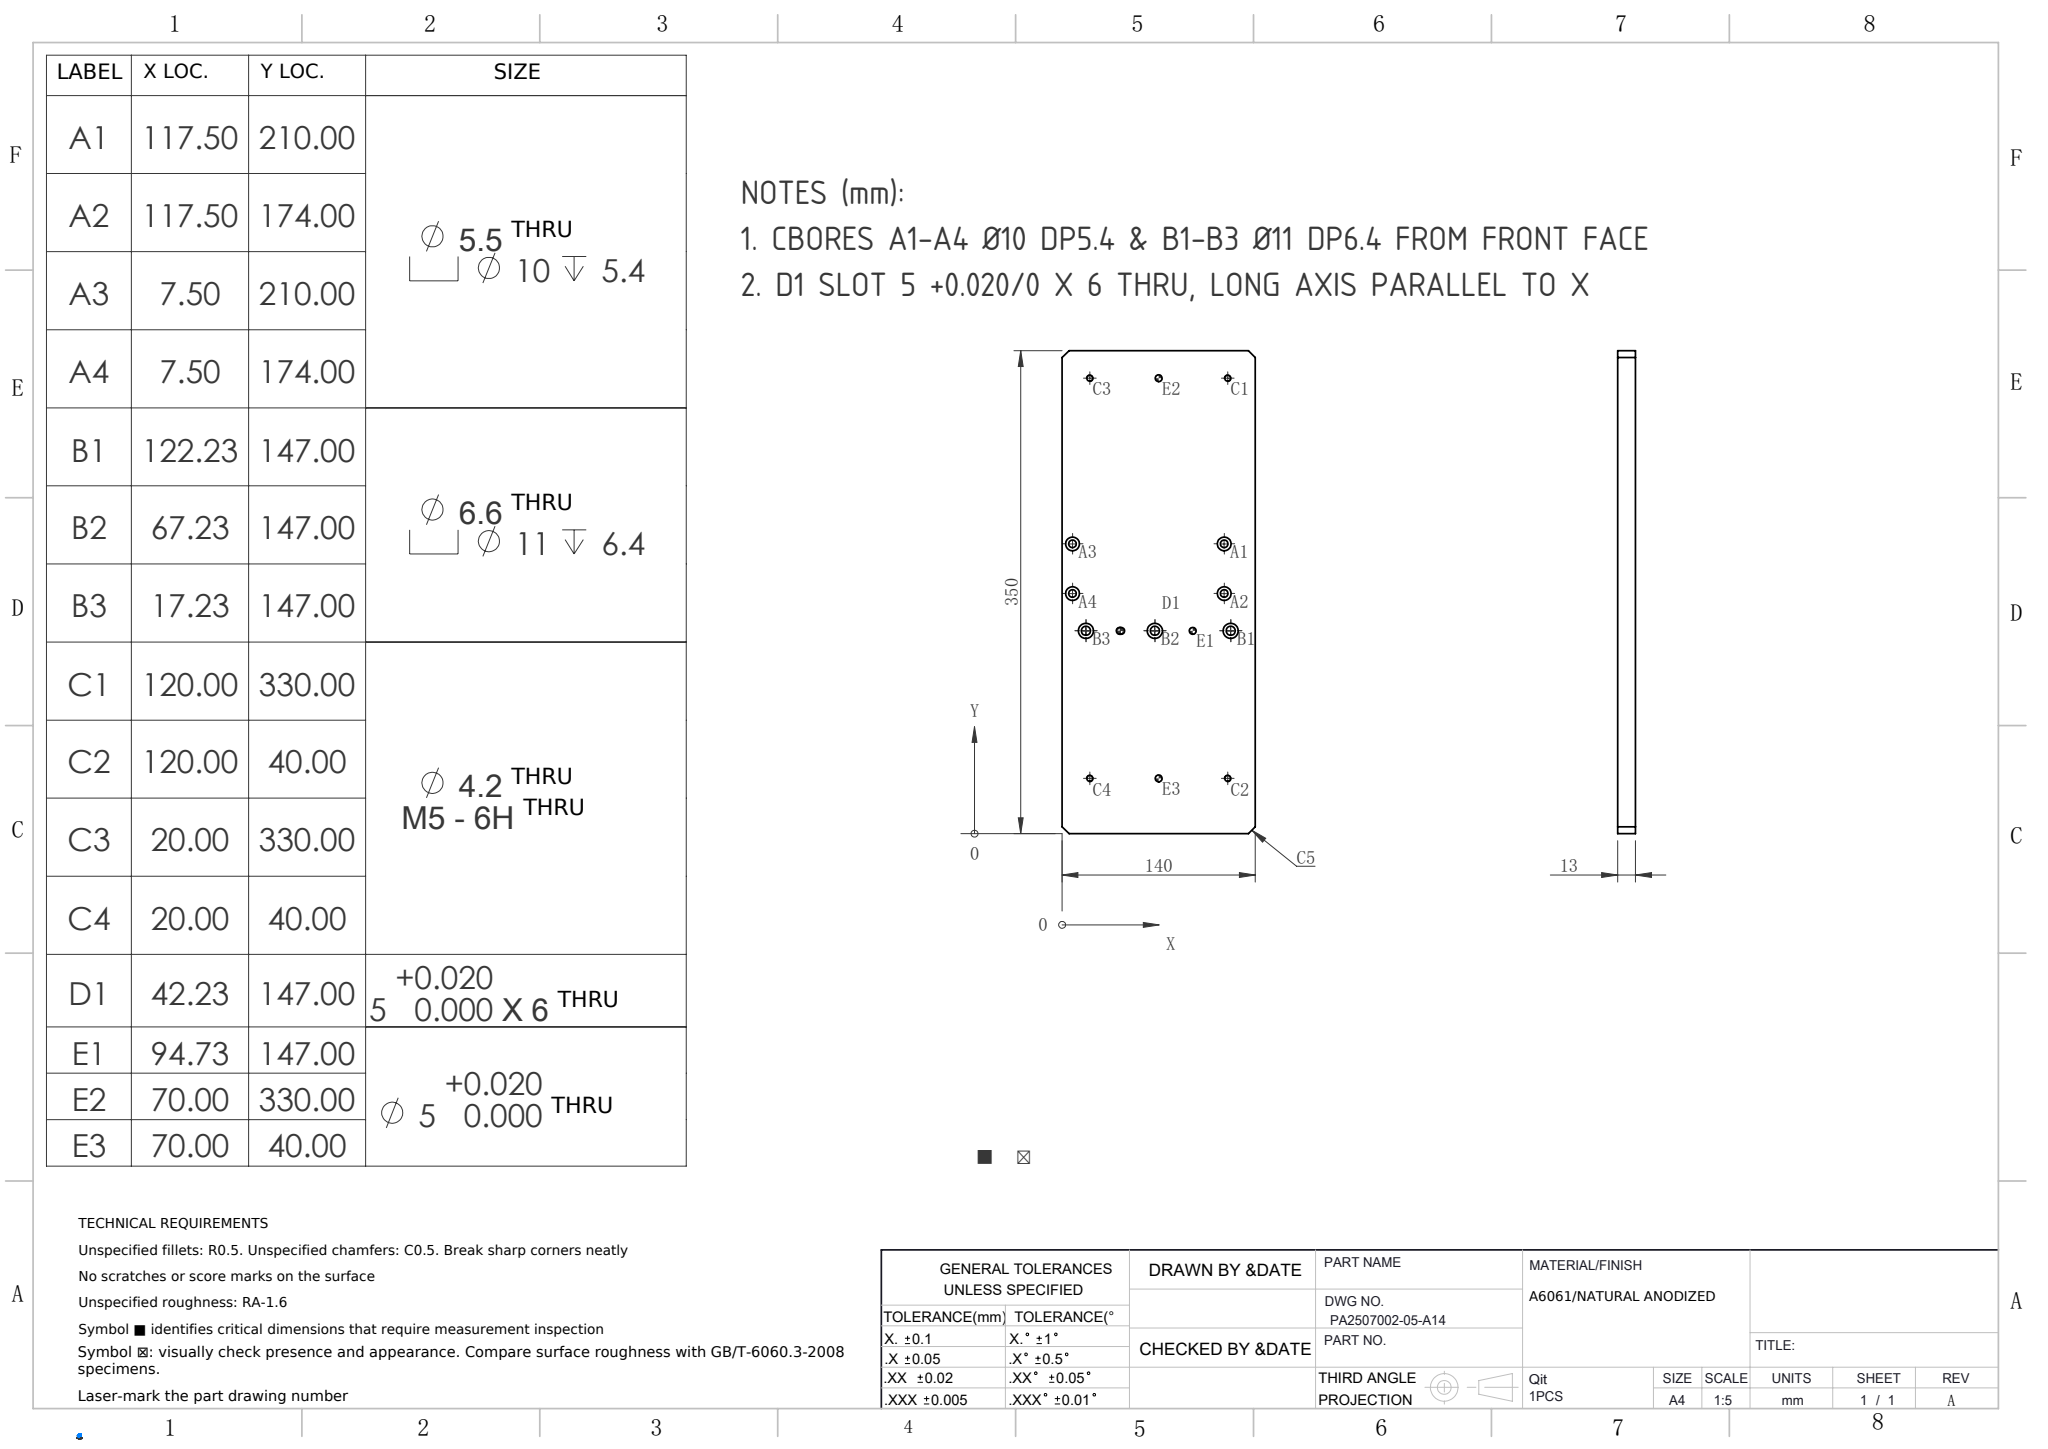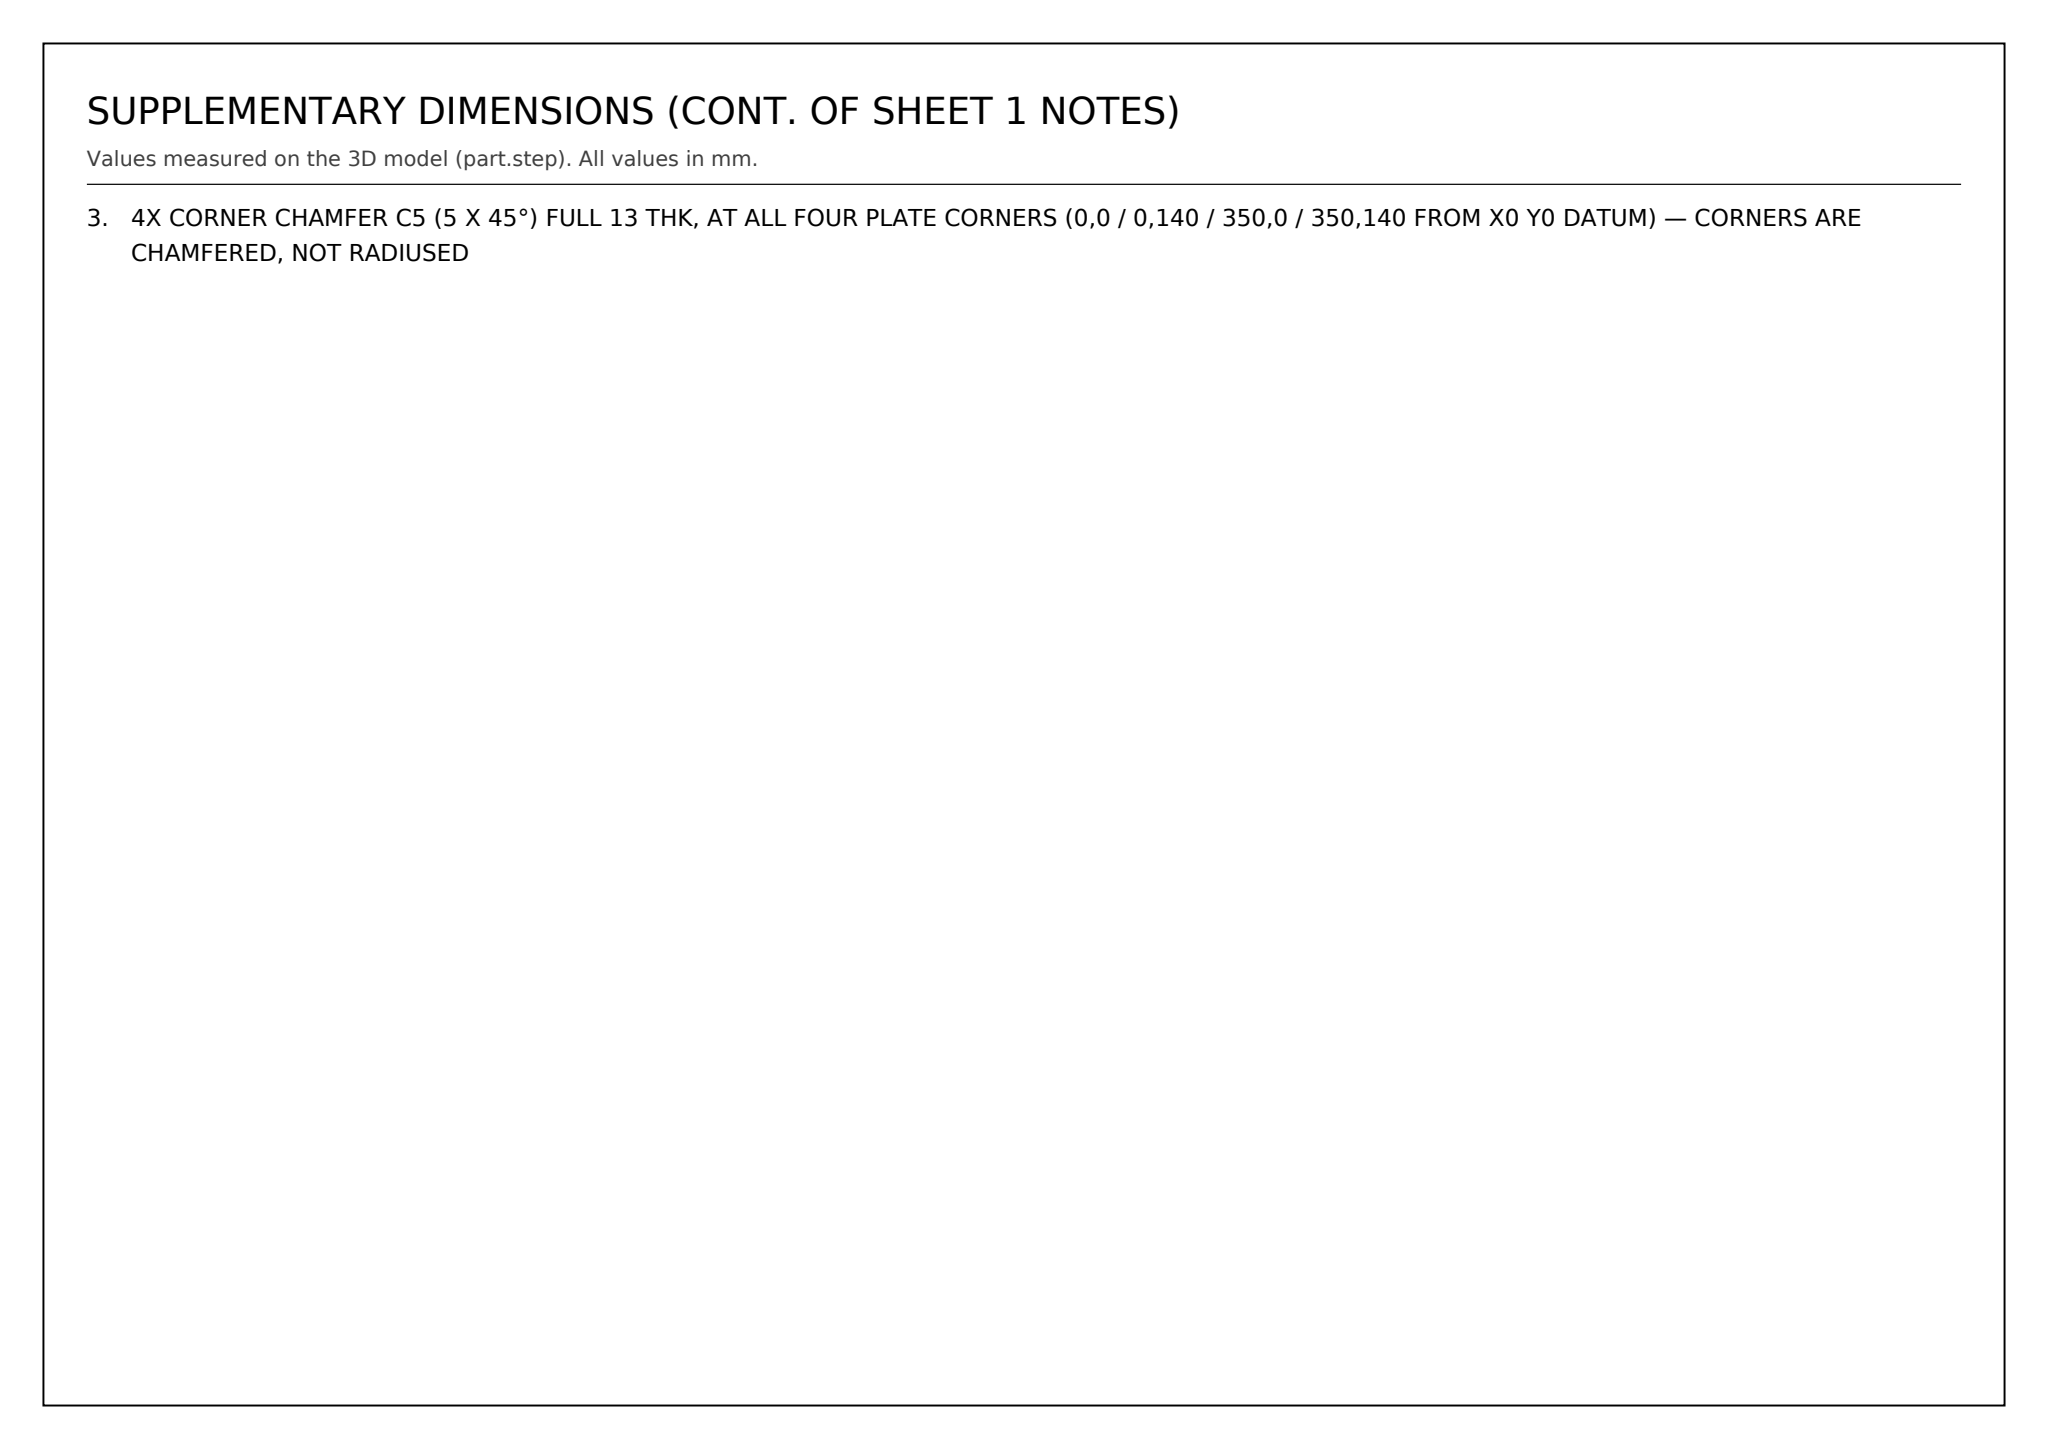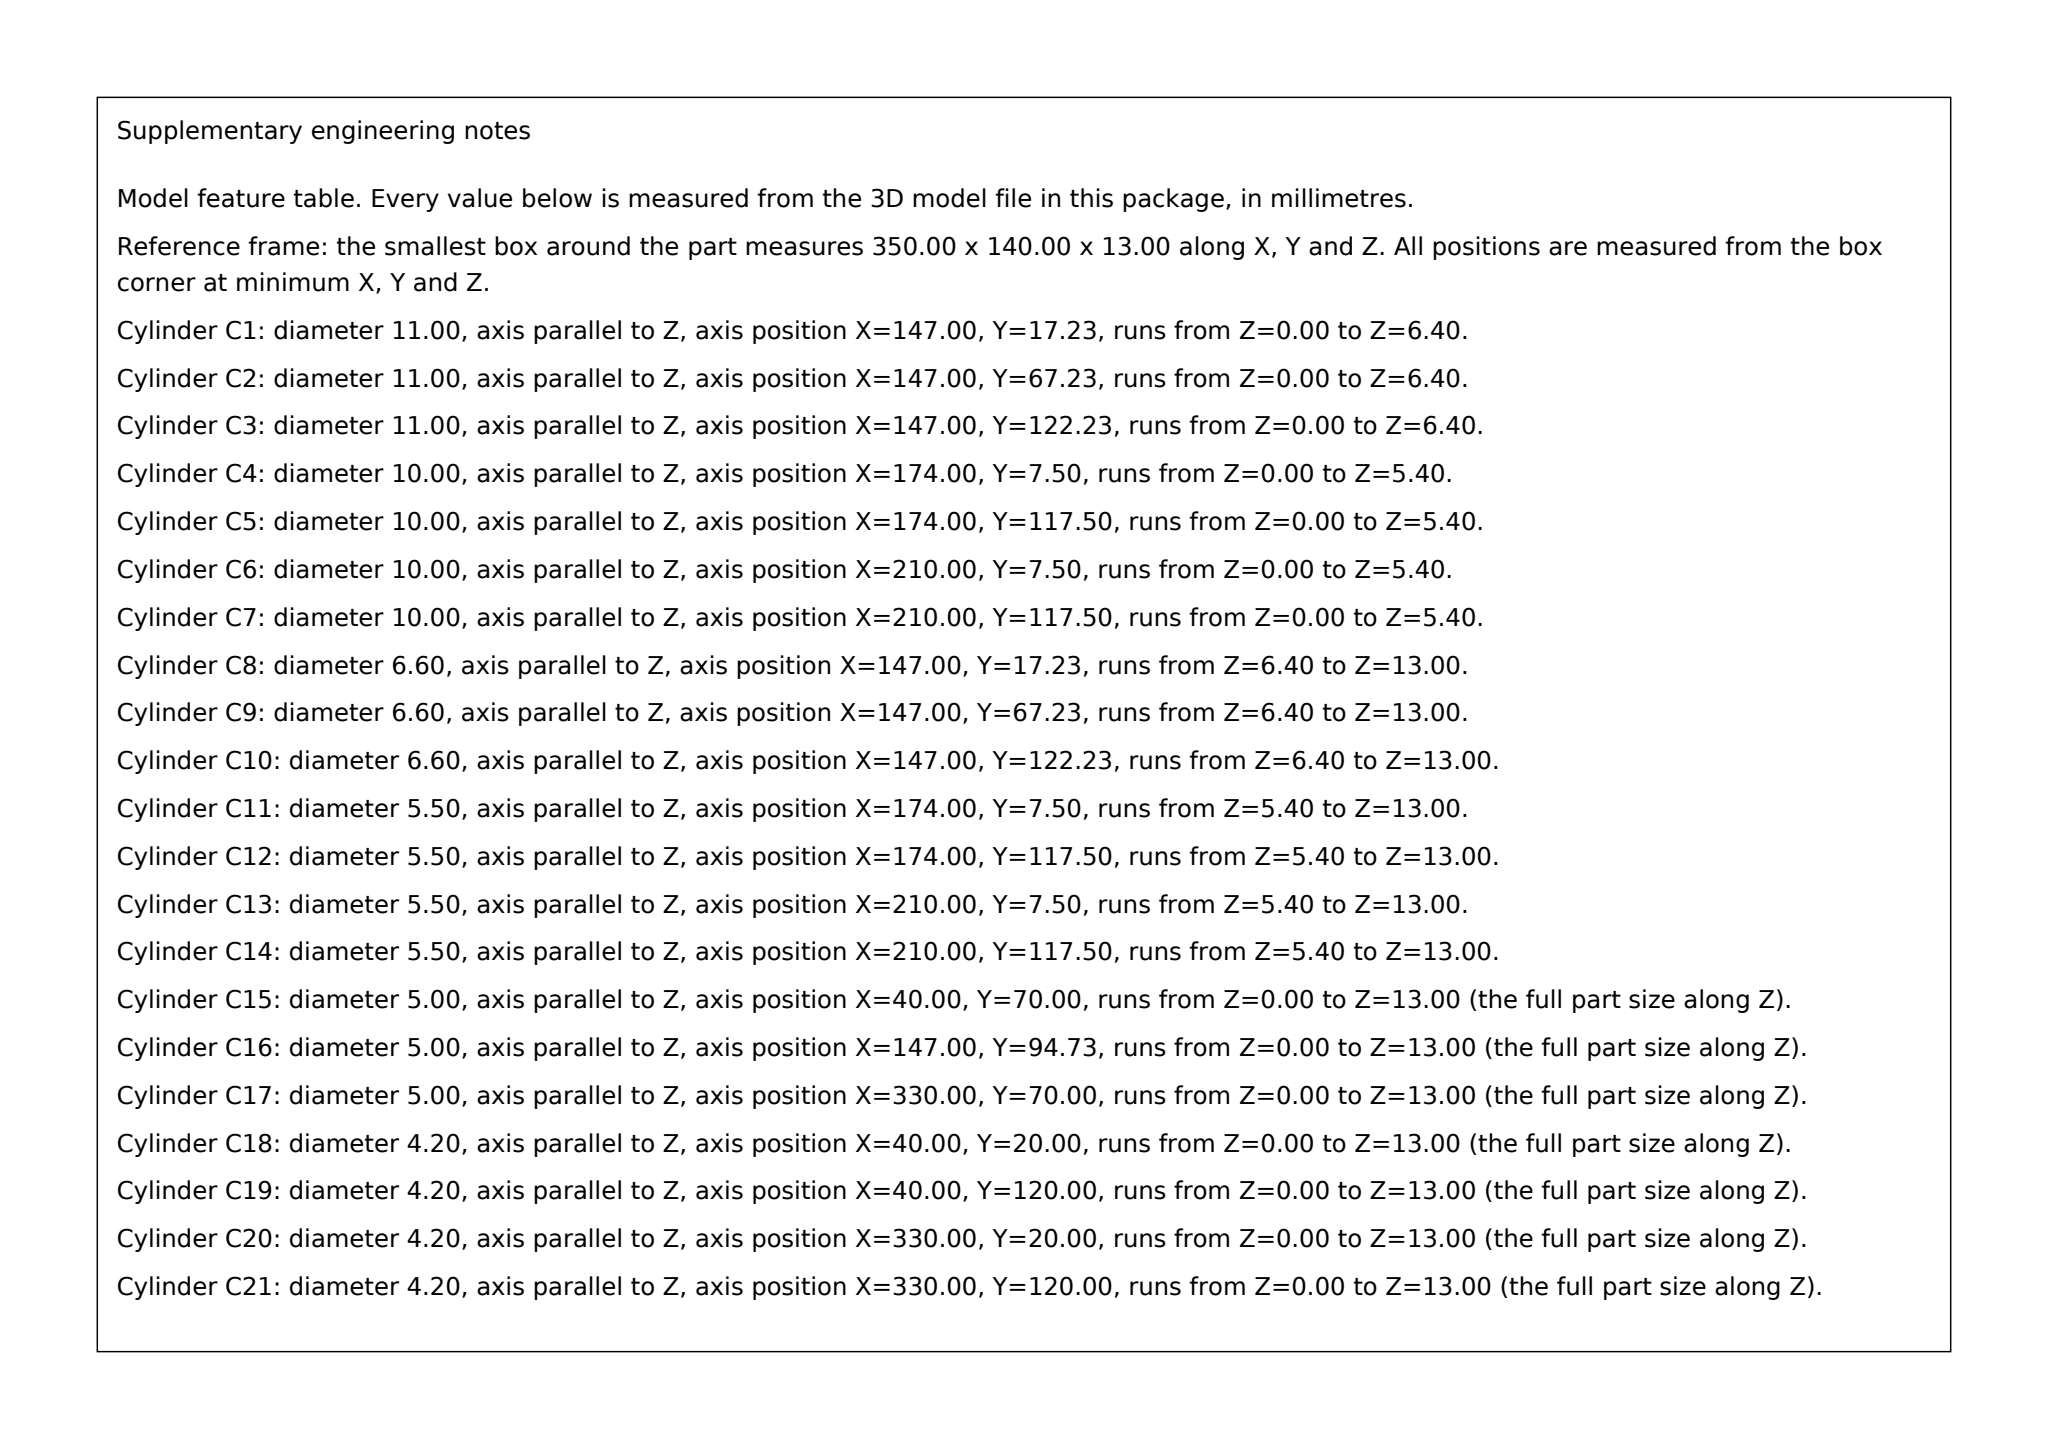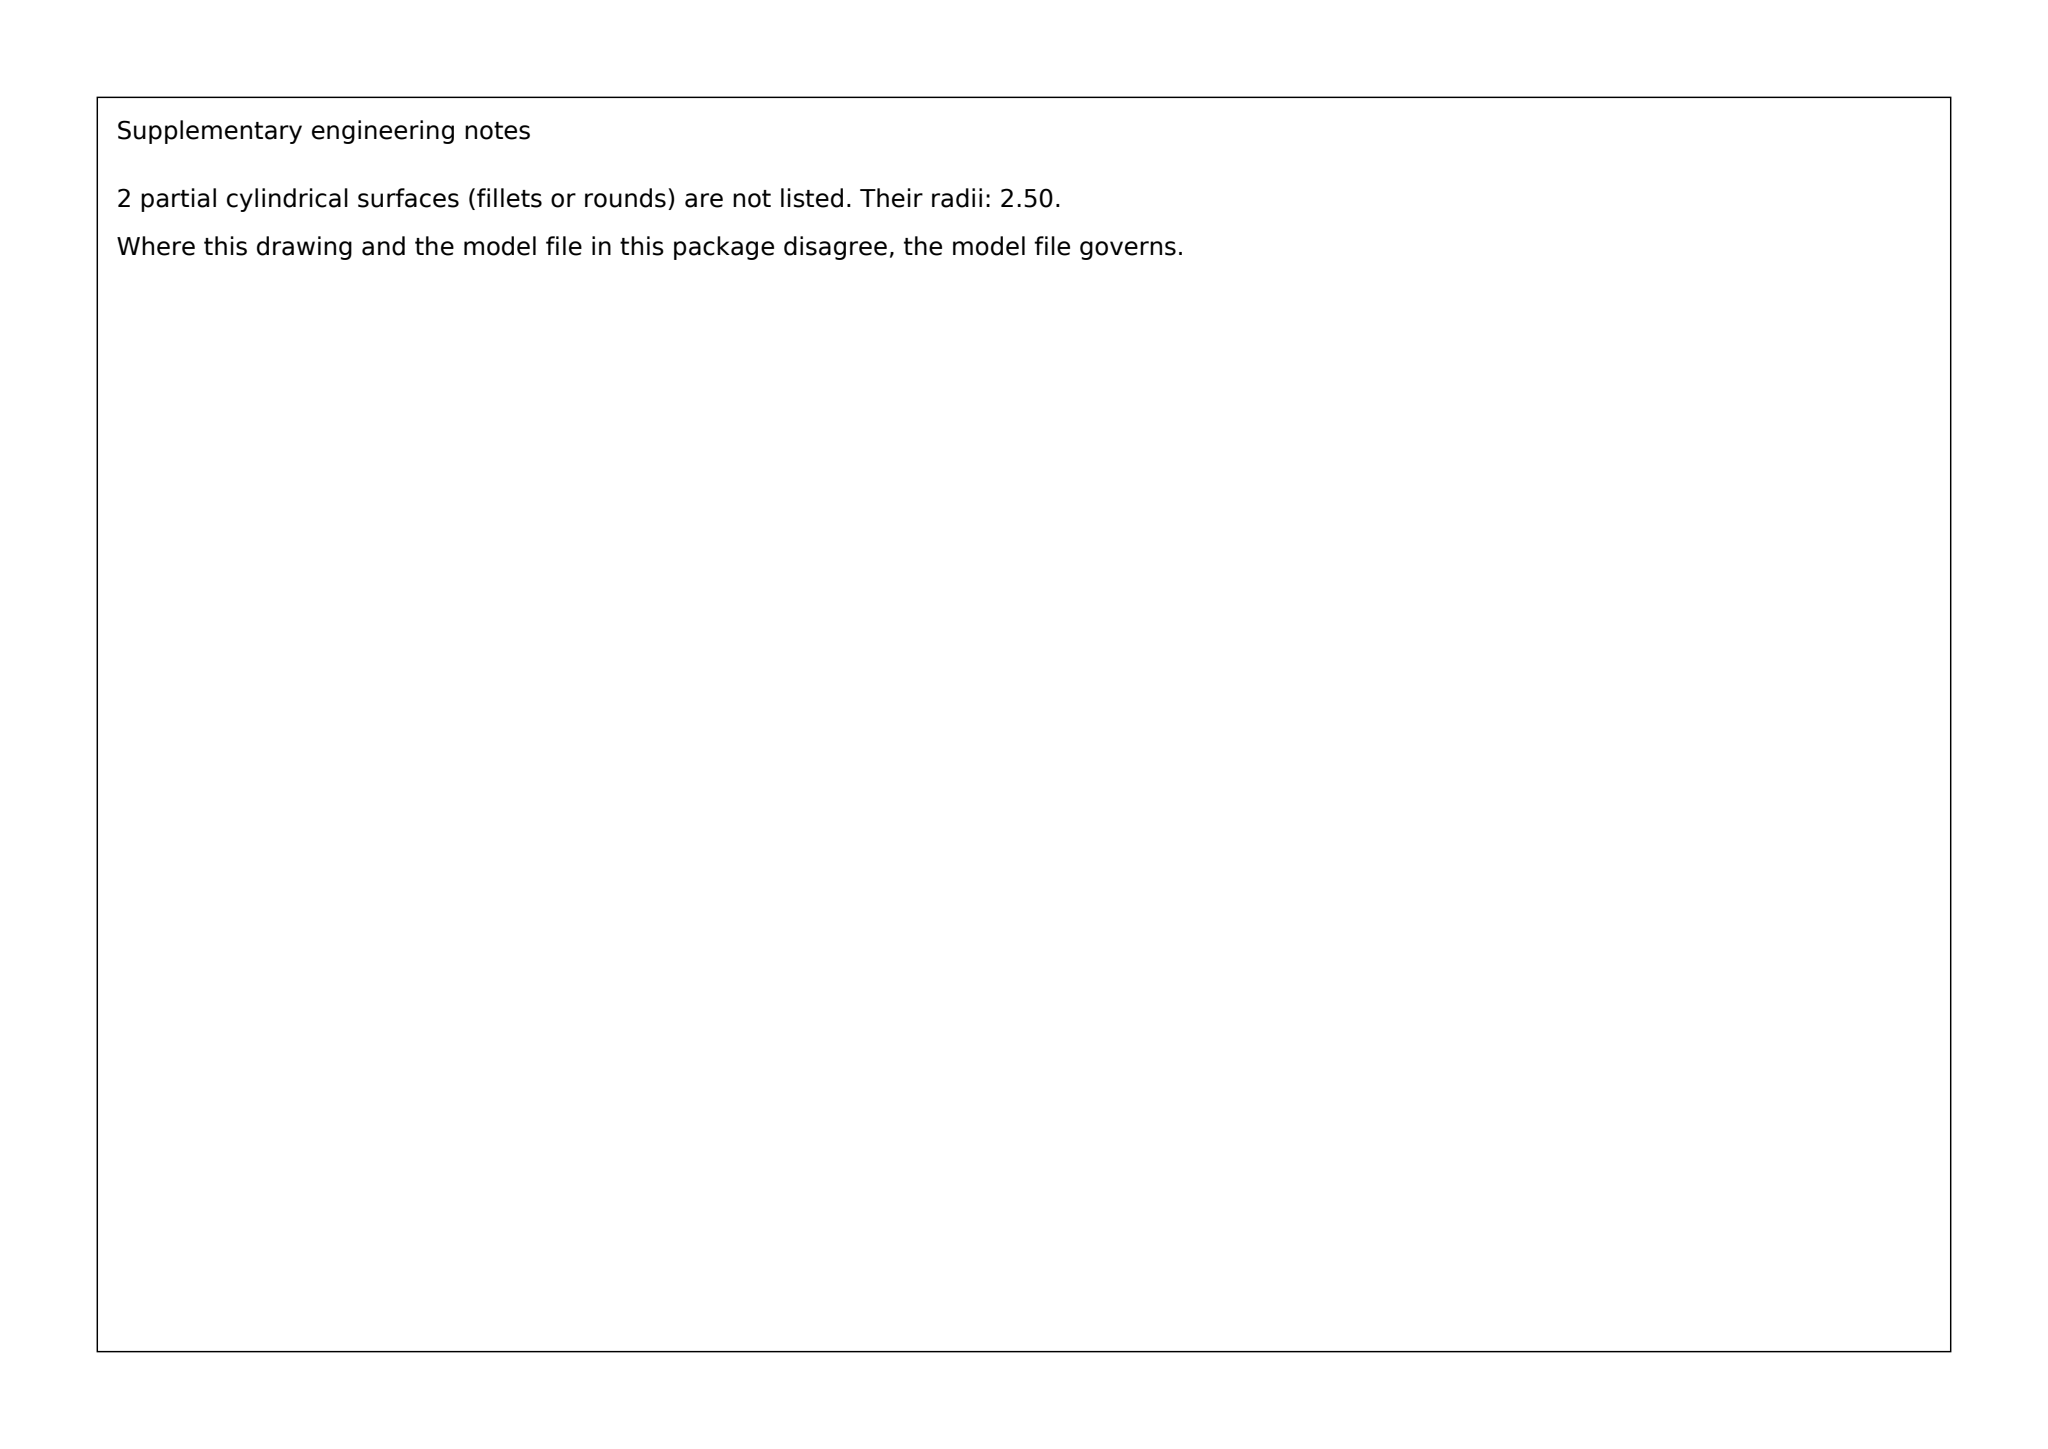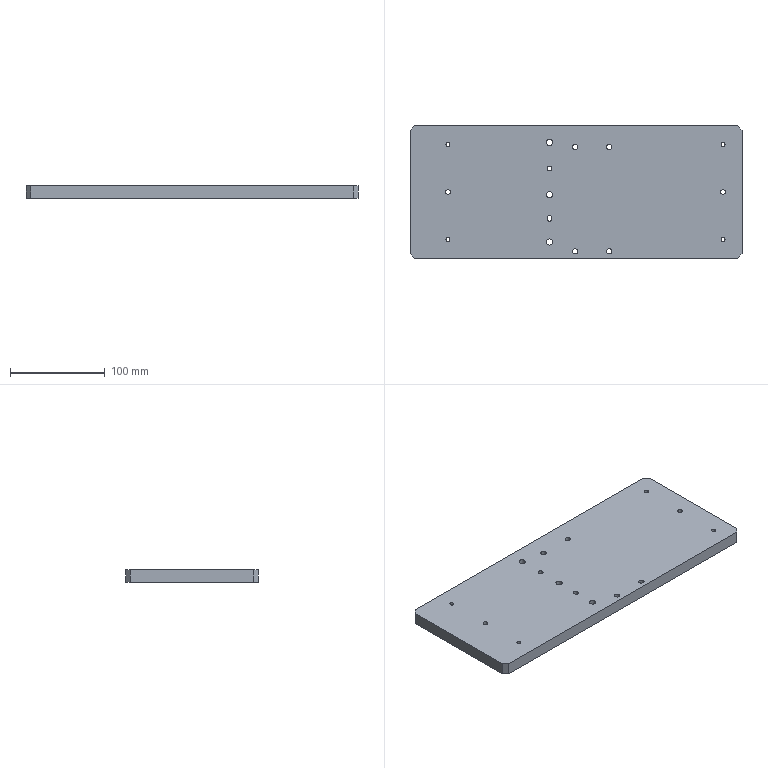Part | SolidWorks | mm | 1 solid | 63 faces | box 350 x 140 x 13 mm | volume 629623 mm3 | cylinder 44 | plane 19 | commonest cylinder face diameters 10 x8 5.5 x8 5 x8 4.2 x8 11 x6 6.6 x6
Drawing notes:
CBORES A1-A4 Ø10 DP5.4 & B1-B3 Ø11 DP6.4 FROM FRONT FACE | from the solid: Ø10 c'bore floors at z=5.4 (4x), Ø11 floors at z=6.4 (3x) from z=0 face; Ø5.5 thru length 7.6 = 13-5.4, all from same side of 13 thk plate
D1 SLOT 5 +0.020/0 X 6 THRU, LONG AXIS PARALLEL TO X | from the solid: Two Ø5 z-cyls at model (147,41.73) & (147,42.73), 1.0 apart along model Y = drawing X; side planes x=144.5/149.5 give 5 wide, 6 long slot
4X CORNER CHAMFER C5 (5 X 45°) FULL 13 THK, AT ALL FOUR PLATE CORNERS (0,0 / 0,140 / 350,0 / 350,140 FROM X0 Y0 DATUM) — CORNERS ARE CHAMFERED, NOT RADIUSED | from the solid: inclined_planes: four 45.0/45.0/90.0 faces, size [5.0,5.0,13.0], bbox_from [0,0,0], [0,135,0], [345,0,0], [345,135,0]